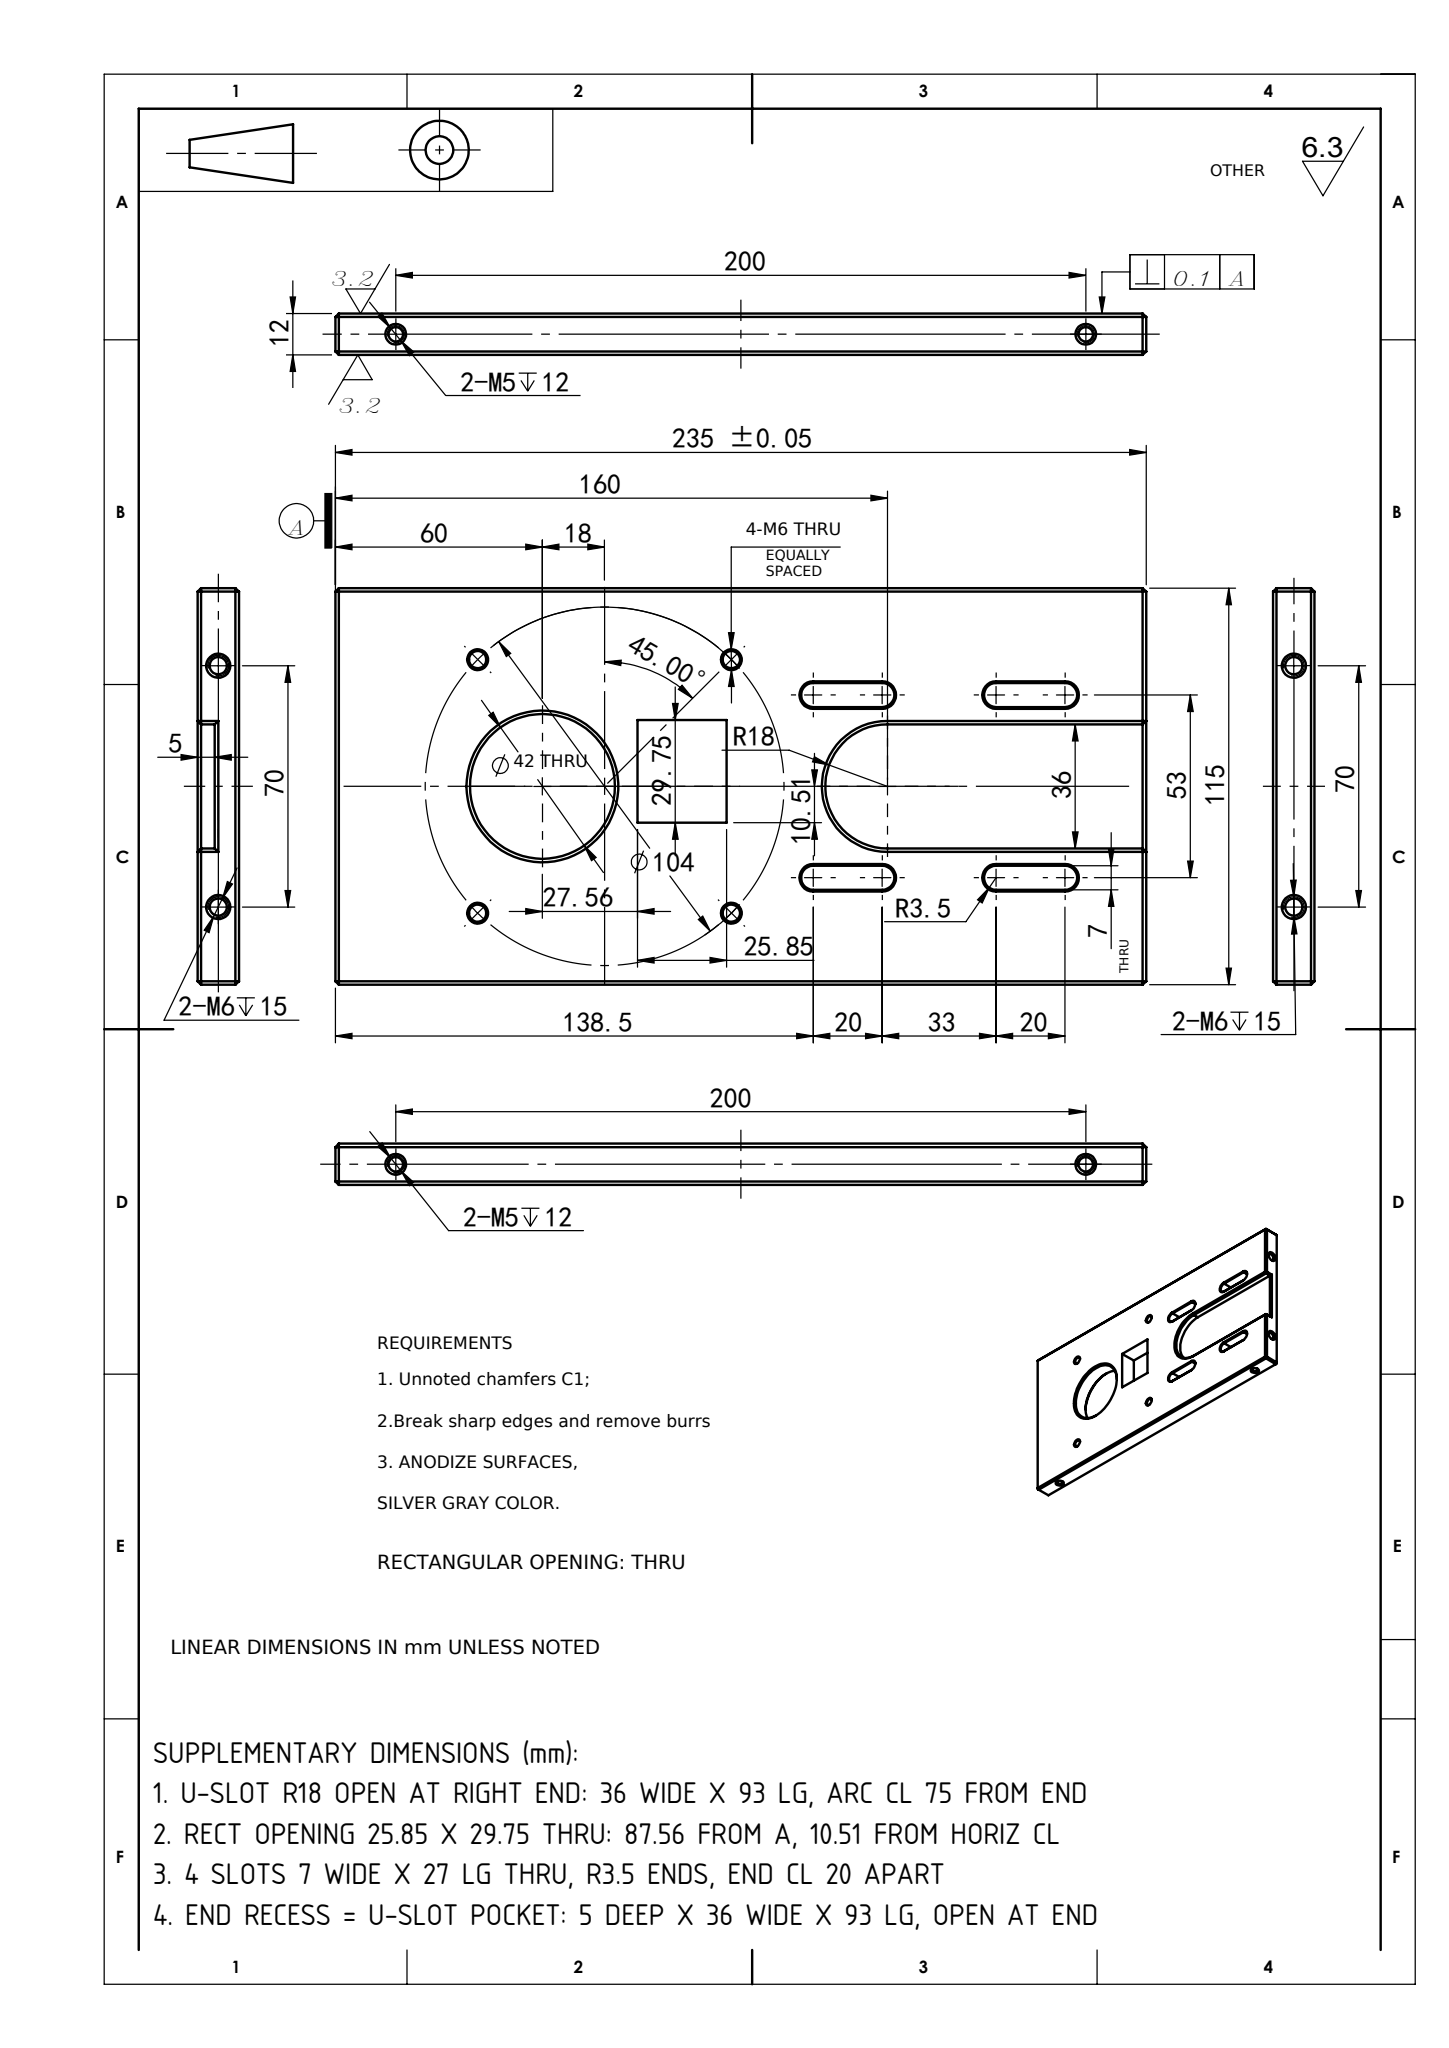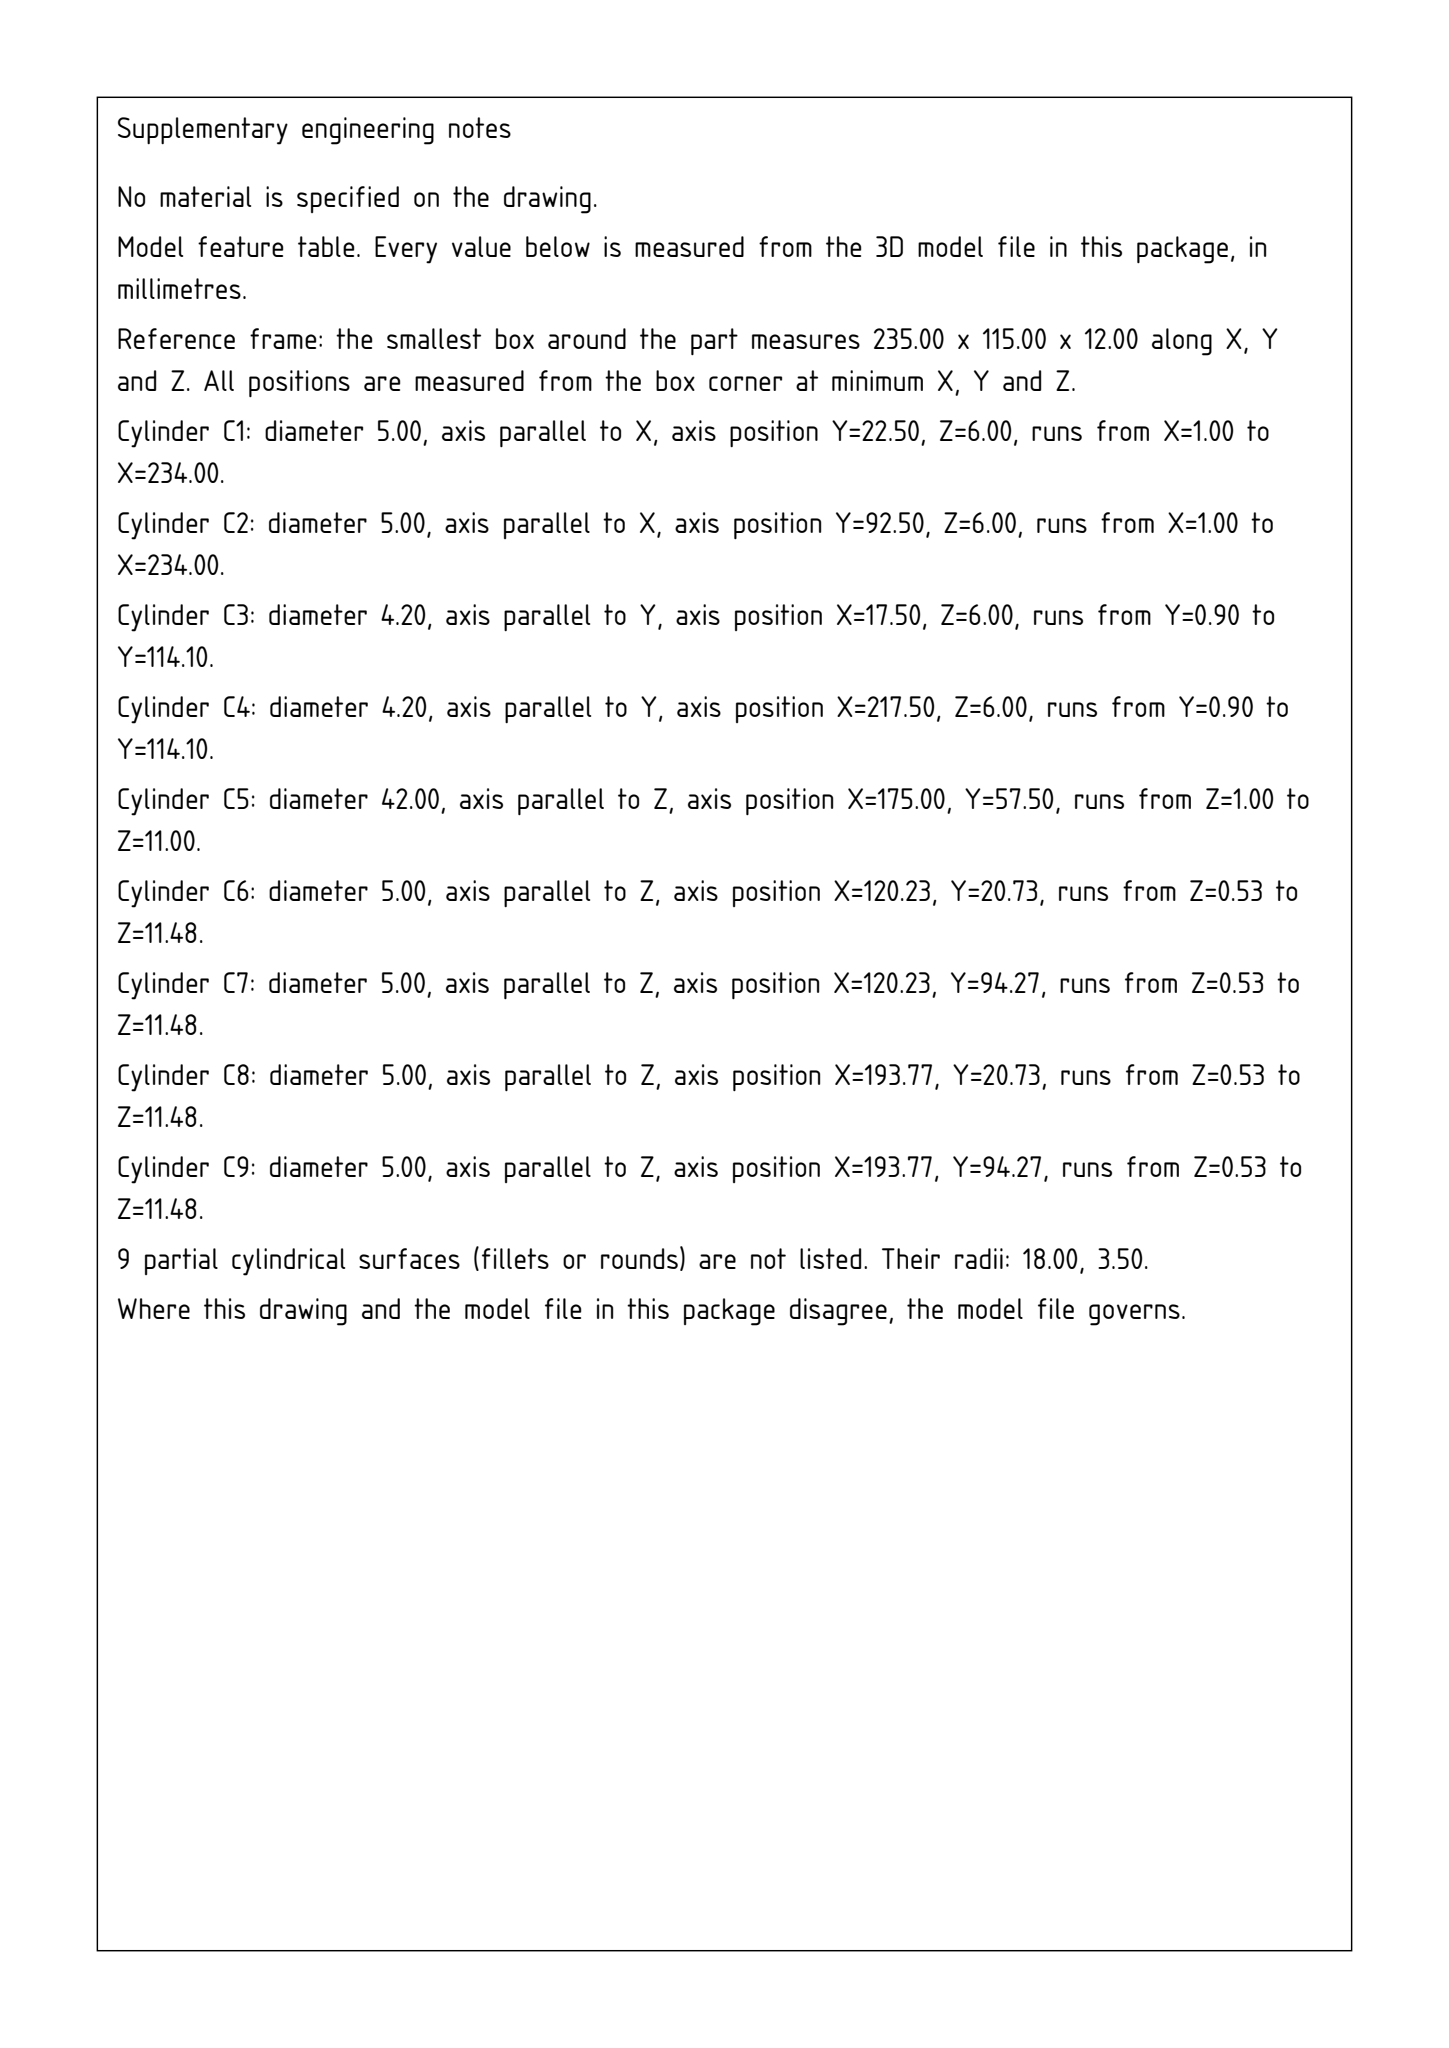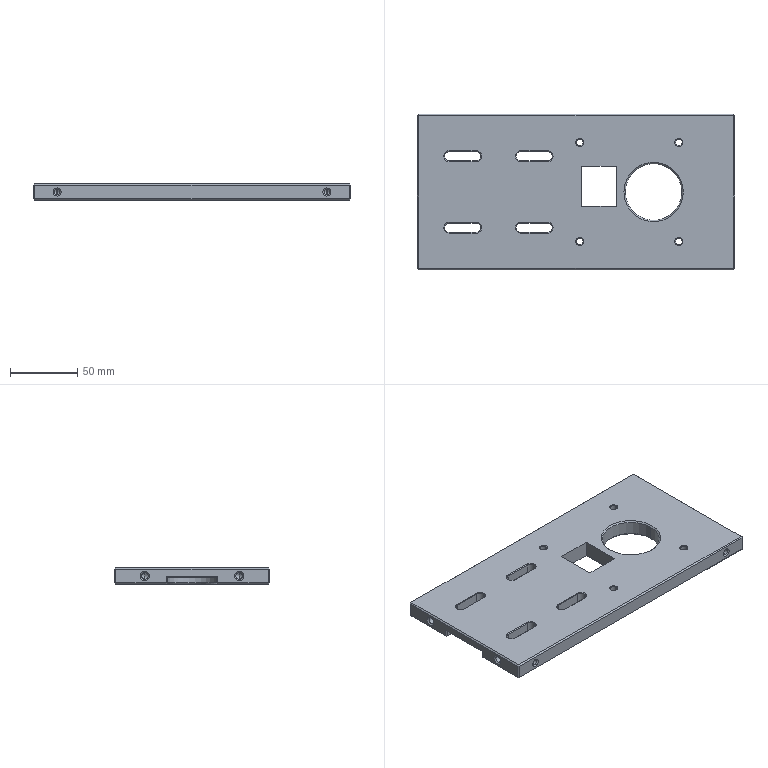Part | SolidWorks | mm | 1 solid | 181 faces | box 235 x 115 x 12 mm | volume 269270 mm3 | cone 77 | plane 65 | cylinder 39 | commonest cylinder face diameters 5 x16 7 x12 4.2 x8 42 x2 36 x1
build123d program:
from build123d import *

# Parameters (mm, degrees)
SKETCH1_W                  = 235
SKETCH1_H                  = 115
SKETCH1_R                  = 21
EXTRUDE1_DEPTH             = 6
CUT_EXTRUDE2_DEPTH         = 5
CHAMFER1_SIZE              = 1
M6_TAPPED_HOLE2_AT_2_COUNT = 2
M6_TAPPED_HOLE2_AT_2_PITCH = 73.539
M6_TAPPED_HOLE2_AT_3_COUNT = 2
M6_TAPPED_HOLE2_AT_3_PITCH = 104
M6_TAPPED_HOLE2_AT_4_COUNT = 2
M6_TAPPED_HOLE2_AT_4_PITCH = 73.539
M6_TAPPED_HOLE1_AT_2_COUNT = 2
M6_TAPPED_HOLE1_AT_2_PITCH = 70
M5_TAPPED_HOLE1_AT_2_COUNT = 2
M5_TAPPED_HOLE1_AT_2_PITCH = 200
CUT_EXTRUDE1_DEPTH         = 132.364
CHAMFER2_SIZE              = 0.5
SKETCH14_W                 = 25.847
SKETCH14_H                 = 29.752
CUT_EXTRUDE3_DEPTH         = 62


with BuildPart() as part:
    # Sketch1 → Extrude1 (new, symmetric)
    with BuildSketch(Plane.XY):
        Rectangle(SKETCH1_W, SKETCH1_H)
        with Locations((57.5, 0)):
            Circle(SKETCH1_R, mode=Mode.SUBTRACT)
    extrude(amount=EXTRUDE1_DEPTH, both=True)

    # Sketch13 → Cut-Extrude2 (cut)
    with BuildSketch(Plane.XY.offset(-6)):
        with BuildLine():
            Line((-42.5, 18), (-117.5, 18))
            Line((-117.5, 18), (-117.5, -18))
            Line((-117.5, -18), (-42.5, -18))
            ThreePointArc((-42.5, -18), (-24.5, 0), (-42.5, 18))
        make_face()
    extrude(amount=CUT_EXTRUDE2_DEPTH, mode=Mode.SUBTRACT)

    # Chamfer1
    chamfer1_edges = [part.edges().sort_by_distance(p)[0] for p in [
        (117.5, 0, 6),
        (36.5, 0, -6),
        (36.5, 0, 6),
        (0, 57.5, 6),
        (-117.5, -37.75, -6),
        (-24.5, 0, -6),
        (-80, 18, -6),
        (-117.5, 18, -3.5),
        (-80, -18, -6),
        (-117.5, -18, -3.5),
        (-117.5, 0, -1),
        (-117.5, 0, 6),
        (0, 57.5, -6),
        (117.5, 0, -6),
        (0, -57.5, -6),
        (-117.5, 37.75, -6),
        (0, -57.5, 6),
        (-117.5, 57.5, 0),
        (117.5, 57.5, 0),
        (117.5, -57.5, 0),
        (-117.5, -57.5, 0),
    ]]
    chamfer(chamfer1_edges, length=CHAMFER1_SIZE)

    # Sketch4 → M6 Tapped Hole2 (revolve, cut)
    with BuildSketch(Plane(origin=(2.73, 36.77, 6), x_dir=(0, -1, 0), z_dir=(1, 0, 0))):
        Polygon((0, 0), (0, 12), (3.025, 12), (2.5, 11.475), (2.5, 0.525), (3.025, 0), align=None)
    m6_tapped_hole2 = revolve(axis=Axis((2.73, 36.77, 12.35), (0, 0, -1)), mode=Mode.SUBTRACT)

    # M6 Tapped Hole2 at 2: M6 Tapped Hole2 ×2
    with Locations(*[(i * M6_TAPPED_HOLE2_AT_2_PITCH, 0, 0) for i in range(1, M6_TAPPED_HOLE2_AT_2_COUNT)]):
        add(m6_tapped_hole2, mode=Mode.SUBTRACT)

    # M6 Tapped Hole2 at 3: M6 Tapped Hole2 ×2
    with Locations(*[Vector(0.7071, -0.7071, 0) * (i * M6_TAPPED_HOLE2_AT_3_PITCH) for i in range(1, M6_TAPPED_HOLE2_AT_3_COUNT)]):
        add(m6_tapped_hole2, mode=Mode.SUBTRACT)

    # M6 Tapped Hole2 at 4: M6 Tapped Hole2 ×2
    with Locations(*[(0, -i * M6_TAPPED_HOLE2_AT_4_PITCH, 0) for i in range(1, M6_TAPPED_HOLE2_AT_4_COUNT)]):
        add(m6_tapped_hole2, mode=Mode.SUBTRACT)

    # Sketch6 → M6 Tapped Hole1 (revolve, cut)
    with BuildSketch(Plane(origin=(-117.5, -35, 0), x_dir=(0, 0, 1), z_dir=(0, 1, 0))):
        Polygon((0, 0), (0, 21.502), (2.5, 20), (2.5, 1), (3.5, 0), align=None)
    m6_tapped_hole1 = revolve(axis=Axis((-123.85, -35, 0), (1, 0, 0)), mode=Mode.SUBTRACT)

    # M6 Tapped Hole1 at 2: M6 Tapped Hole1 ×2
    with Locations(*[(0, i * M6_TAPPED_HOLE1_AT_2_PITCH, 0) for i in range(1, M6_TAPPED_HOLE1_AT_2_COUNT)]):
        add(m6_tapped_hole1, mode=Mode.SUBTRACT)

    # Sketch8 → M5 Tapped Hole1 (revolve, cut)
    with BuildSketch(Plane(origin=(100, 57.5, 0), x_dir=(0, 0, 1), z_dir=(1, 0, 0))):
        Polygon((0, 0), (0, 17.262), (2.1, 16), (2.1, 0.9), (3, 0), align=None)
    m5_tapped_hole1 = revolve(axis=Axis((100, 63.85, 0), (0, -1, 0)), mode=Mode.SUBTRACT)

    # M5 Tapped Hole1 at 2: M5 Tapped Hole1 ×2
    with Locations(*[(-i * M5_TAPPED_HOLE1_AT_2_PITCH, 0, 0) for i in range(1, M5_TAPPED_HOLE1_AT_2_COUNT)]):
        add(m5_tapped_hole1, mode=Mode.SUBTRACT)

    # Mirror1: M6 Tapped Hole1 across plane
    add(m6_tapped_hole1.mirror(Plane(origin=(0, 0, 0), x_dir=(0, 0, 1), z_dir=(1, 0, 0))), mode=Mode.SUBTRACT)

    # Mirror1 copy 1 sketch → Mirror1 copy 1 (revolve, cut)
    with BuildSketch(Plane(origin=(117.5, 35, 0), x_dir=(0, 0, 1), z_dir=(0, 1, 0))):
        Polygon((0, 0), (0, -21.502), (2.5, -20), (2.5, -1), (3.5, 0), align=None)
    revolve(axis=Axis((123.85, 35, 0), (1, 0, 0)), mode=Mode.SUBTRACT)

    # Mirror2: M5 Tapped Hole1 across plane
    add(m5_tapped_hole1.mirror(Plane.ZX), mode=Mode.SUBTRACT)

    # Mirror2 copy 1 sketch → Mirror2 copy 1 (revolve, cut)
    with BuildSketch(Plane(origin=(-100, -57.5, 0), x_dir=(0, 0, 1), z_dir=(1, 0, 0))):
        Polygon((0, 0), (0, -17.262), (2.1, -16), (2.1, -0.9), (3, 0), align=None)
    revolve(axis=Axis((-100, -63.85, 0), (0, -1, 0)), mode=Mode.SUBTRACT)

    # Sketch12 → Cut-Extrude1 (cut, through all)
    with BuildSketch(Plane.XY.offset(6)):
        with BuildLine():
            Line((-41, 30), (-21, 30))
            ThreePointArc((-21, 30), (-17.5, 26.5), (-21, 23))
            Line((-21, 23), (-41, 23))
            ThreePointArc((-41, 23), (-44.5, 26.5), (-41, 30))
        make_face()
        with BuildLine():
            Line((-94, 30), (-74, 30))
            ThreePointArc((-74, 30), (-70.5, 26.5), (-74, 23))
            Line((-74, 23), (-94, 23))
            ThreePointArc((-94, 23), (-97.5, 26.5), (-94, 30))
        make_face()
        with BuildLine():
            Line((-41, -23), (-21, -23))
            ThreePointArc((-21, -23), (-17.5, -26.5), (-21, -30))
            Line((-21, -30), (-41, -30))
            ThreePointArc((-41, -30), (-44.5, -26.5), (-41, -23))
        make_face()
        with BuildLine():
            Line((-94, -23), (-74, -23))
            ThreePointArc((-74, -23), (-70.5, -26.5), (-74, -30))
            Line((-74, -30), (-94, -30))
            ThreePointArc((-94, -30), (-97.5, -26.5), (-94, -23))
        make_face()
    extrude(amount=-CUT_EXTRUDE1_DEPTH, mode=Mode.SUBTRACT)

    # Chamfer2
    chamfer2_edges = [part.edges().sort_by_distance(p)[0] for p in [
        (-44.5, 26.5, -6),
        (-31, 30, -6),
        (-17.5, 26.5, -6),
        (-31, 23, -6),
        (-44.5, 26.5, 6),
        (-31, 23, 6),
        (-17.5, 26.5, 6),
        (-31, 30, 6),
        (-97.5, 26.5, -6),
        (-84, 30, -6),
        (-70.5, 26.5, -6),
        (-84, 23, -6),
        (-97.5, 26.5, 6),
        (-84, 23, 6),
        (-70.5, 26.5, 6),
        (-84, 30, 6),
        (-44.5, -26.5, -6),
        (-31, -23, -6),
        (-17.5, -26.5, -6),
        (-31, -30, -6),
        (-44.5, -26.5, 6),
        (-31, -30, 6),
        (-17.5, -26.5, 6),
        (-31, -23, 6),
        (-97.5, -26.5, -6),
        (-84, -23, -6),
        (-70.5, -26.5, -6),
        (-84, -30, -6),
        (-97.5, -26.5, 6),
        (-84, -30, 6),
        (-70.5, -26.5, 6),
        (-84, -23, 6),
    ]]
    chamfer(chamfer2_edges, length=CHAMFER2_SIZE)

    # Sketch14 → Cut-Extrude3 (cut)
    with BuildSketch(Plane.XY.offset(6)):
        with Locations((17.014, 4.37)):
            Rectangle(SKETCH14_W, SKETCH14_H)
    extrude(amount=-CUT_EXTRUDE3_DEPTH, mode=Mode.SUBTRACT)


solid = part.part